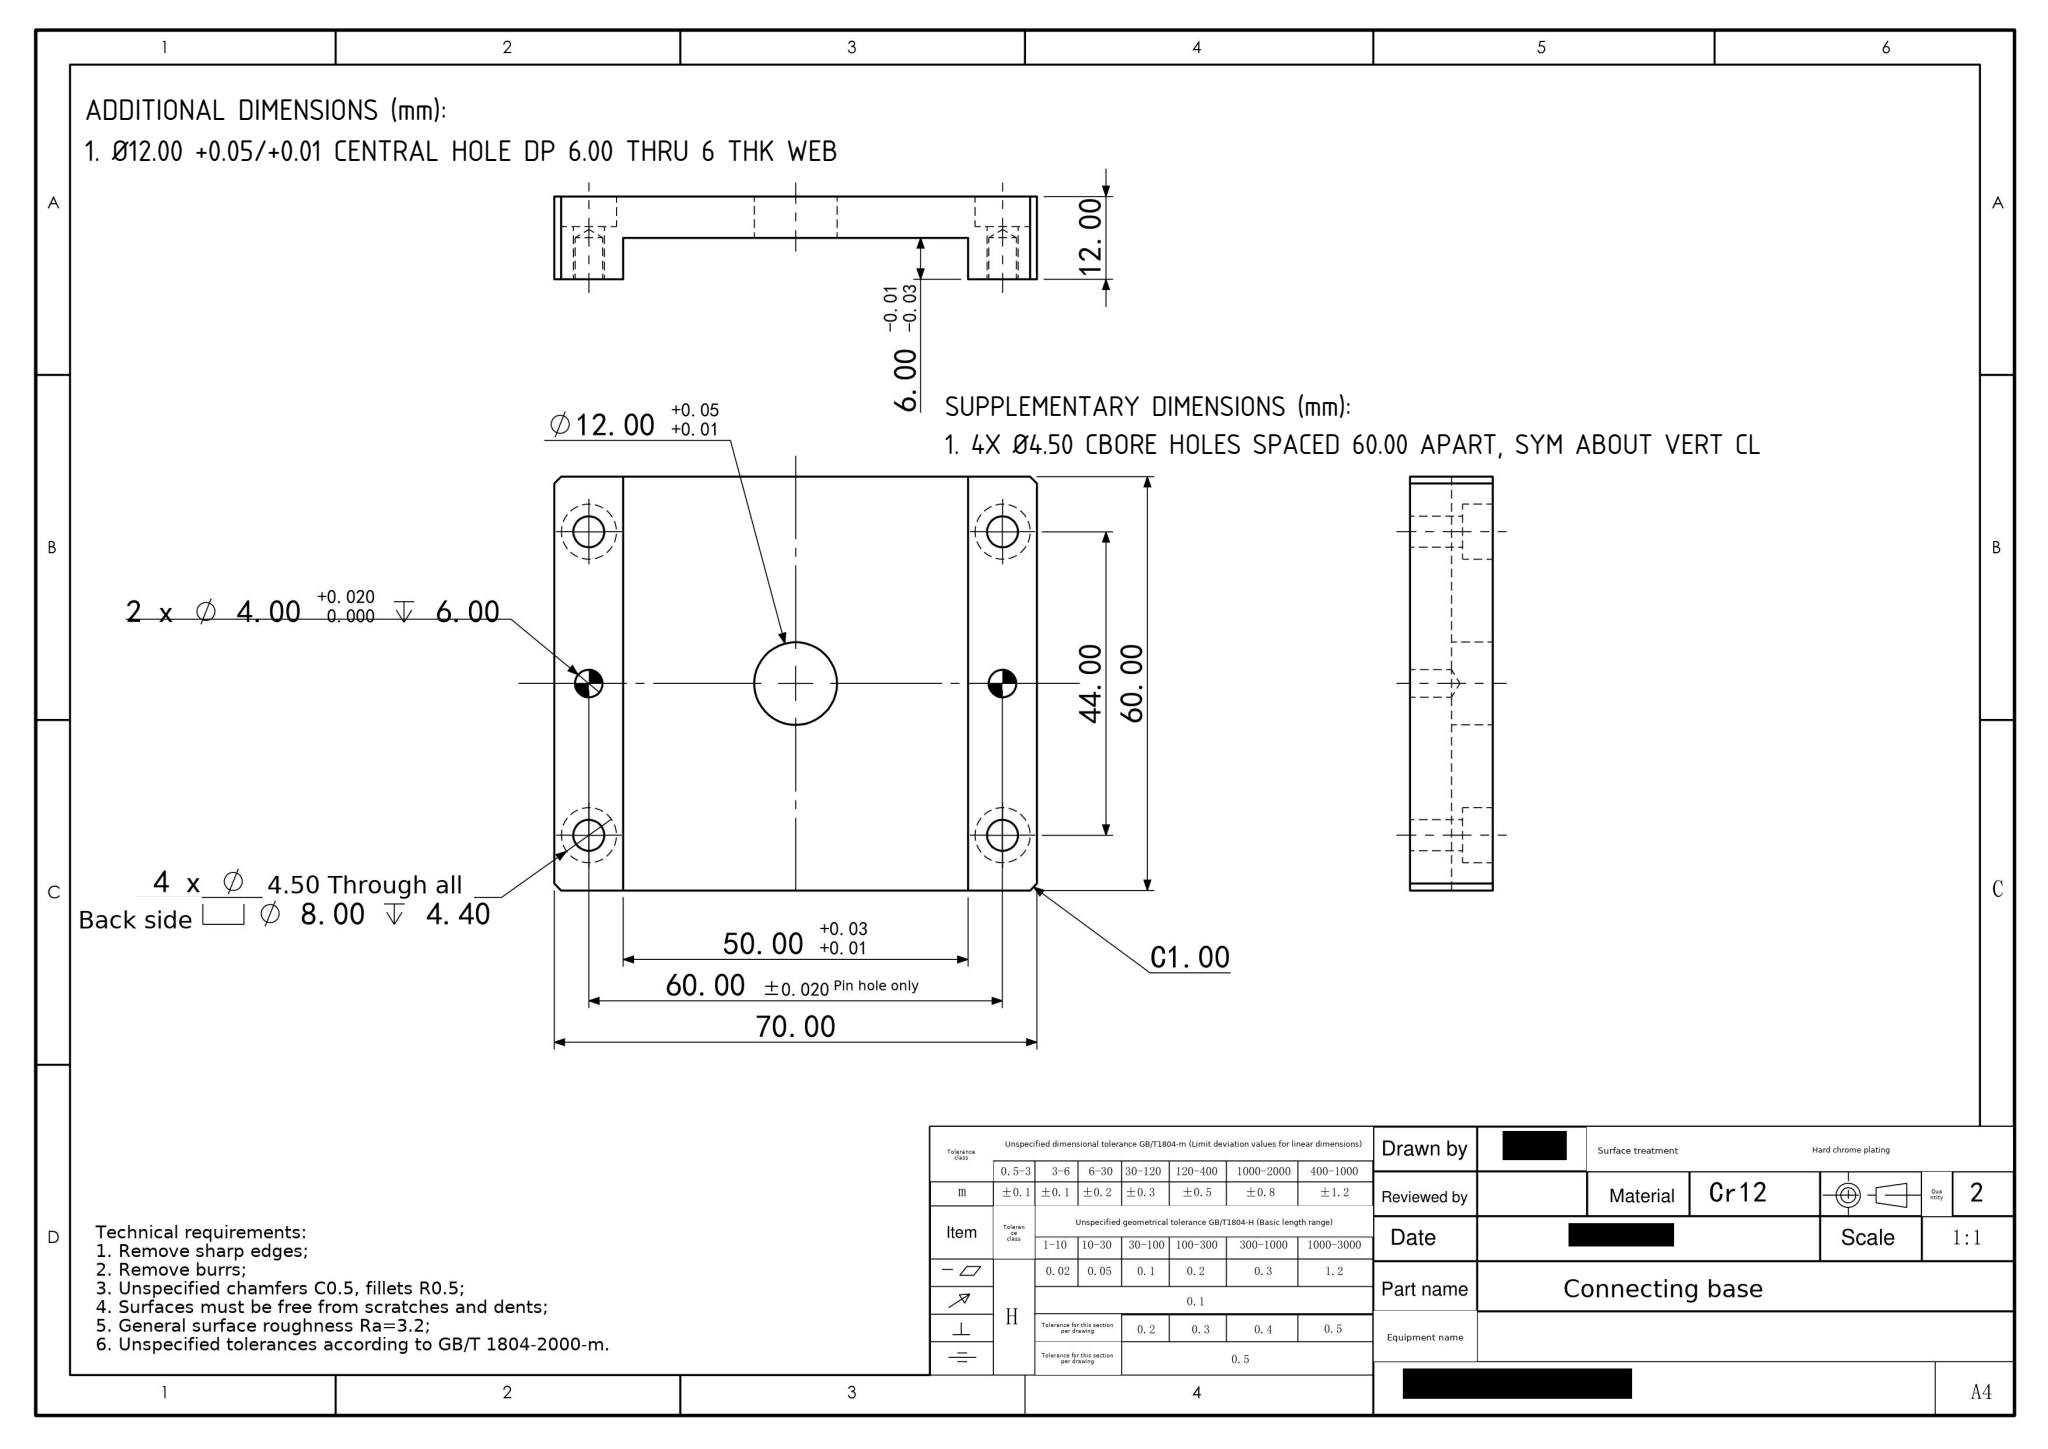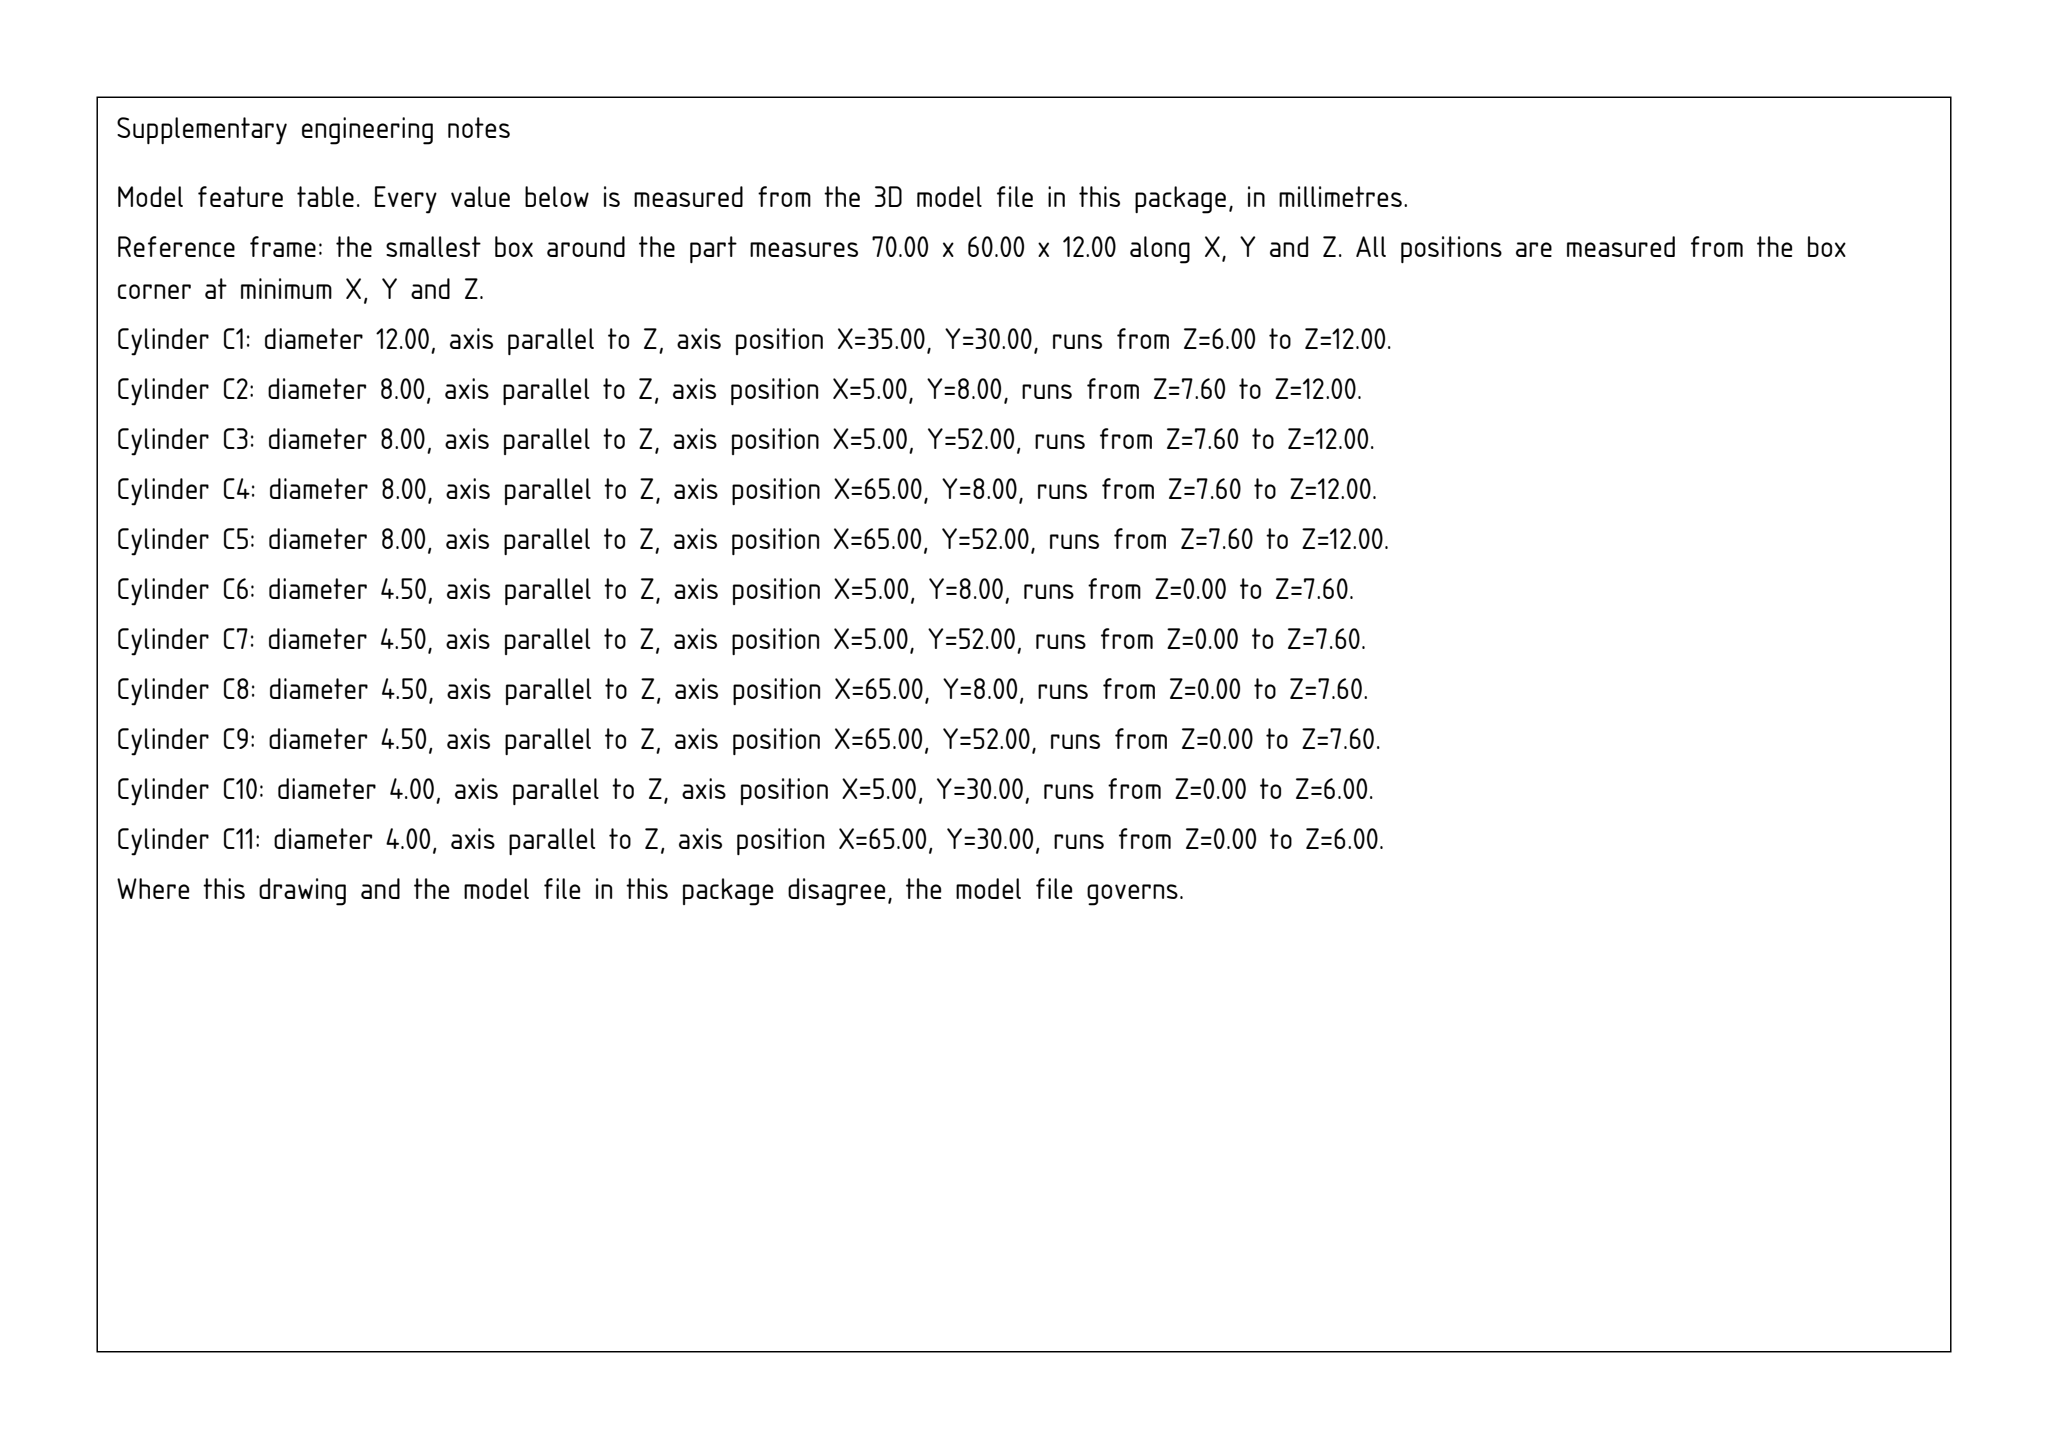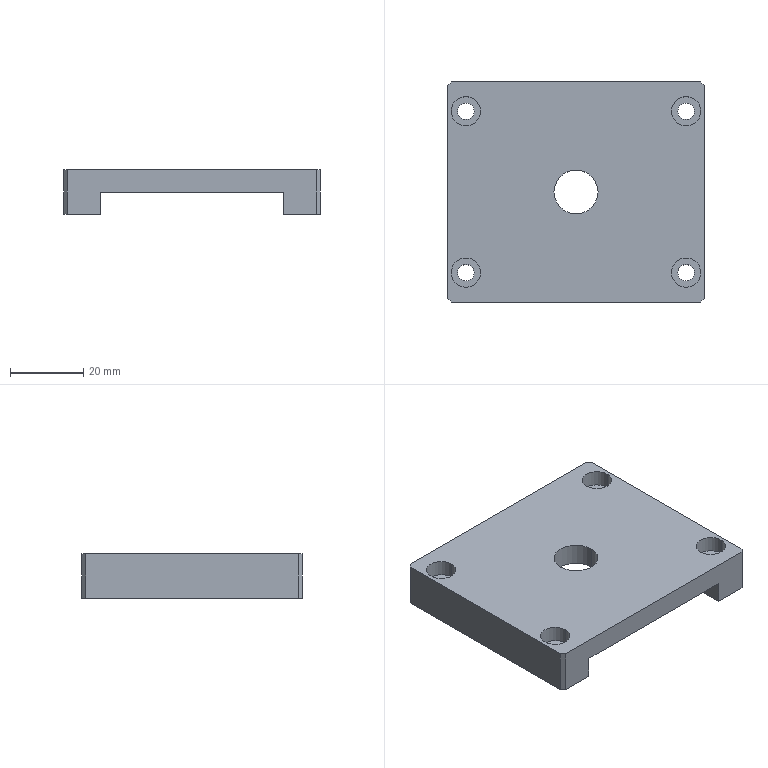Part | SolidWorks | mm | 1 solid | 44 faces | box 70 x 60 x 12 mm | volume 30168 mm3 | cylinder 22 | plane 18 | cone 4 | commonest cylinder face diameters 8 x8 4.5 x8 4 x4 12 x2
build123d program:
from build123d import *

# Parameters (mm, degrees)
SKETCH1_W                                       = 70
SKETCH1_H                                       = 60
BOSS_EXTRUDE1_DEPTH                             = 12
CHAMFER1_SIZE                                   = 1
SKETCH2_W                                       = 50
SKETCH2_H                                       = 120
CUT_EXTRUDE1_DEPTH                              = 6
M4_HEX_SOCKET_HEAD_CAP_SCREW_CBORE1_D           = 4.5
M4_HEX_SOCKET_HEAD_CAP_SCREW_CBORE1_CBORE_D     = 8
M4_HEX_SOCKET_HEAD_CAP_SCREW_CBORE1_CBORE_DEPTH = 4.4
F_4_0MM_DOWEL_PIN_HOLE1_D                       = 4
F_4_0MM_DOWEL_PIN_HOLE1_DEPTH                   = 6
F_4_0MM_DOWEL_PIN_HOLE1_TIP                     = 1.202
SKETCH7_R                                       = 6
CUT_EXTRUDE2_DEPTH                              = 48.634


with BuildPart() as part:
    # Sketch1 → Boss-Extrude1 (new body)
    with BuildSketch(Plane.XY):
        Rectangle(SKETCH1_W, SKETCH1_H)
    extrude(amount=BOSS_EXTRUDE1_DEPTH)

    # Chamfer1
    chamfer1_edges = [part.edges().sort_by_distance(p)[0] for p in [
        (35, -30, 6),
        (-35, -30, 6),
        (-35, 30, 6),
        (35, 30, 6),
    ]]
    chamfer(chamfer1_edges, length=CHAMFER1_SIZE)

    # Sketch2 → Cut-Extrude1 (cut)
    with BuildSketch(Plane(origin=(0, 0, 0), x_dir=(-1, 0, 0), z_dir=(0, 0, -1))):
        with Locations((0, 30)):
            Rectangle(SKETCH2_W, SKETCH2_H)
    extrude(amount=-CUT_EXTRUDE1_DEPTH, mode=Mode.SUBTRACT)

    # M4 Hex Socket Head Cap Screw CBORE1 (through all)
    with Locations(Plane.XY.offset(12)):
        with Locations((-30, -22), (30, -22), (30, 22), (-30, 22)):
            CounterBoreHole(M4_HEX_SOCKET_HEAD_CAP_SCREW_CBORE1_D / 2, M4_HEX_SOCKET_HEAD_CAP_SCREW_CBORE1_CBORE_D / 2, M4_HEX_SOCKET_HEAD_CAP_SCREW_CBORE1_CBORE_DEPTH)

    # 4.0mm Dowel Pin Hole1
    with Locations(Plane(origin=(0, 0, 0), x_dir=(-1, 0, 0), z_dir=(0, 0, -1))):
        with Locations((-30, 0), (30, 0)):
            Hole(F_4_0MM_DOWEL_PIN_HOLE1_D / 2, depth=F_4_0MM_DOWEL_PIN_HOLE1_DEPTH)
            with Locations((0, 0, -(F_4_0MM_DOWEL_PIN_HOLE1_DEPTH + F_4_0MM_DOWEL_PIN_HOLE1_TIP / 2))):  # 118° drill point
                Cone(0, F_4_0MM_DOWEL_PIN_HOLE1_D / 2, F_4_0MM_DOWEL_PIN_HOLE1_TIP, mode=Mode.SUBTRACT)

    # Sketch7 → Cut-Extrude2 (cut, through all)
    with BuildSketch(Plane.XY.offset(12)):
        Circle(SKETCH7_R)
    extrude(amount=-CUT_EXTRUDE2_DEPTH, mode=Mode.SUBTRACT)


solid = part.part